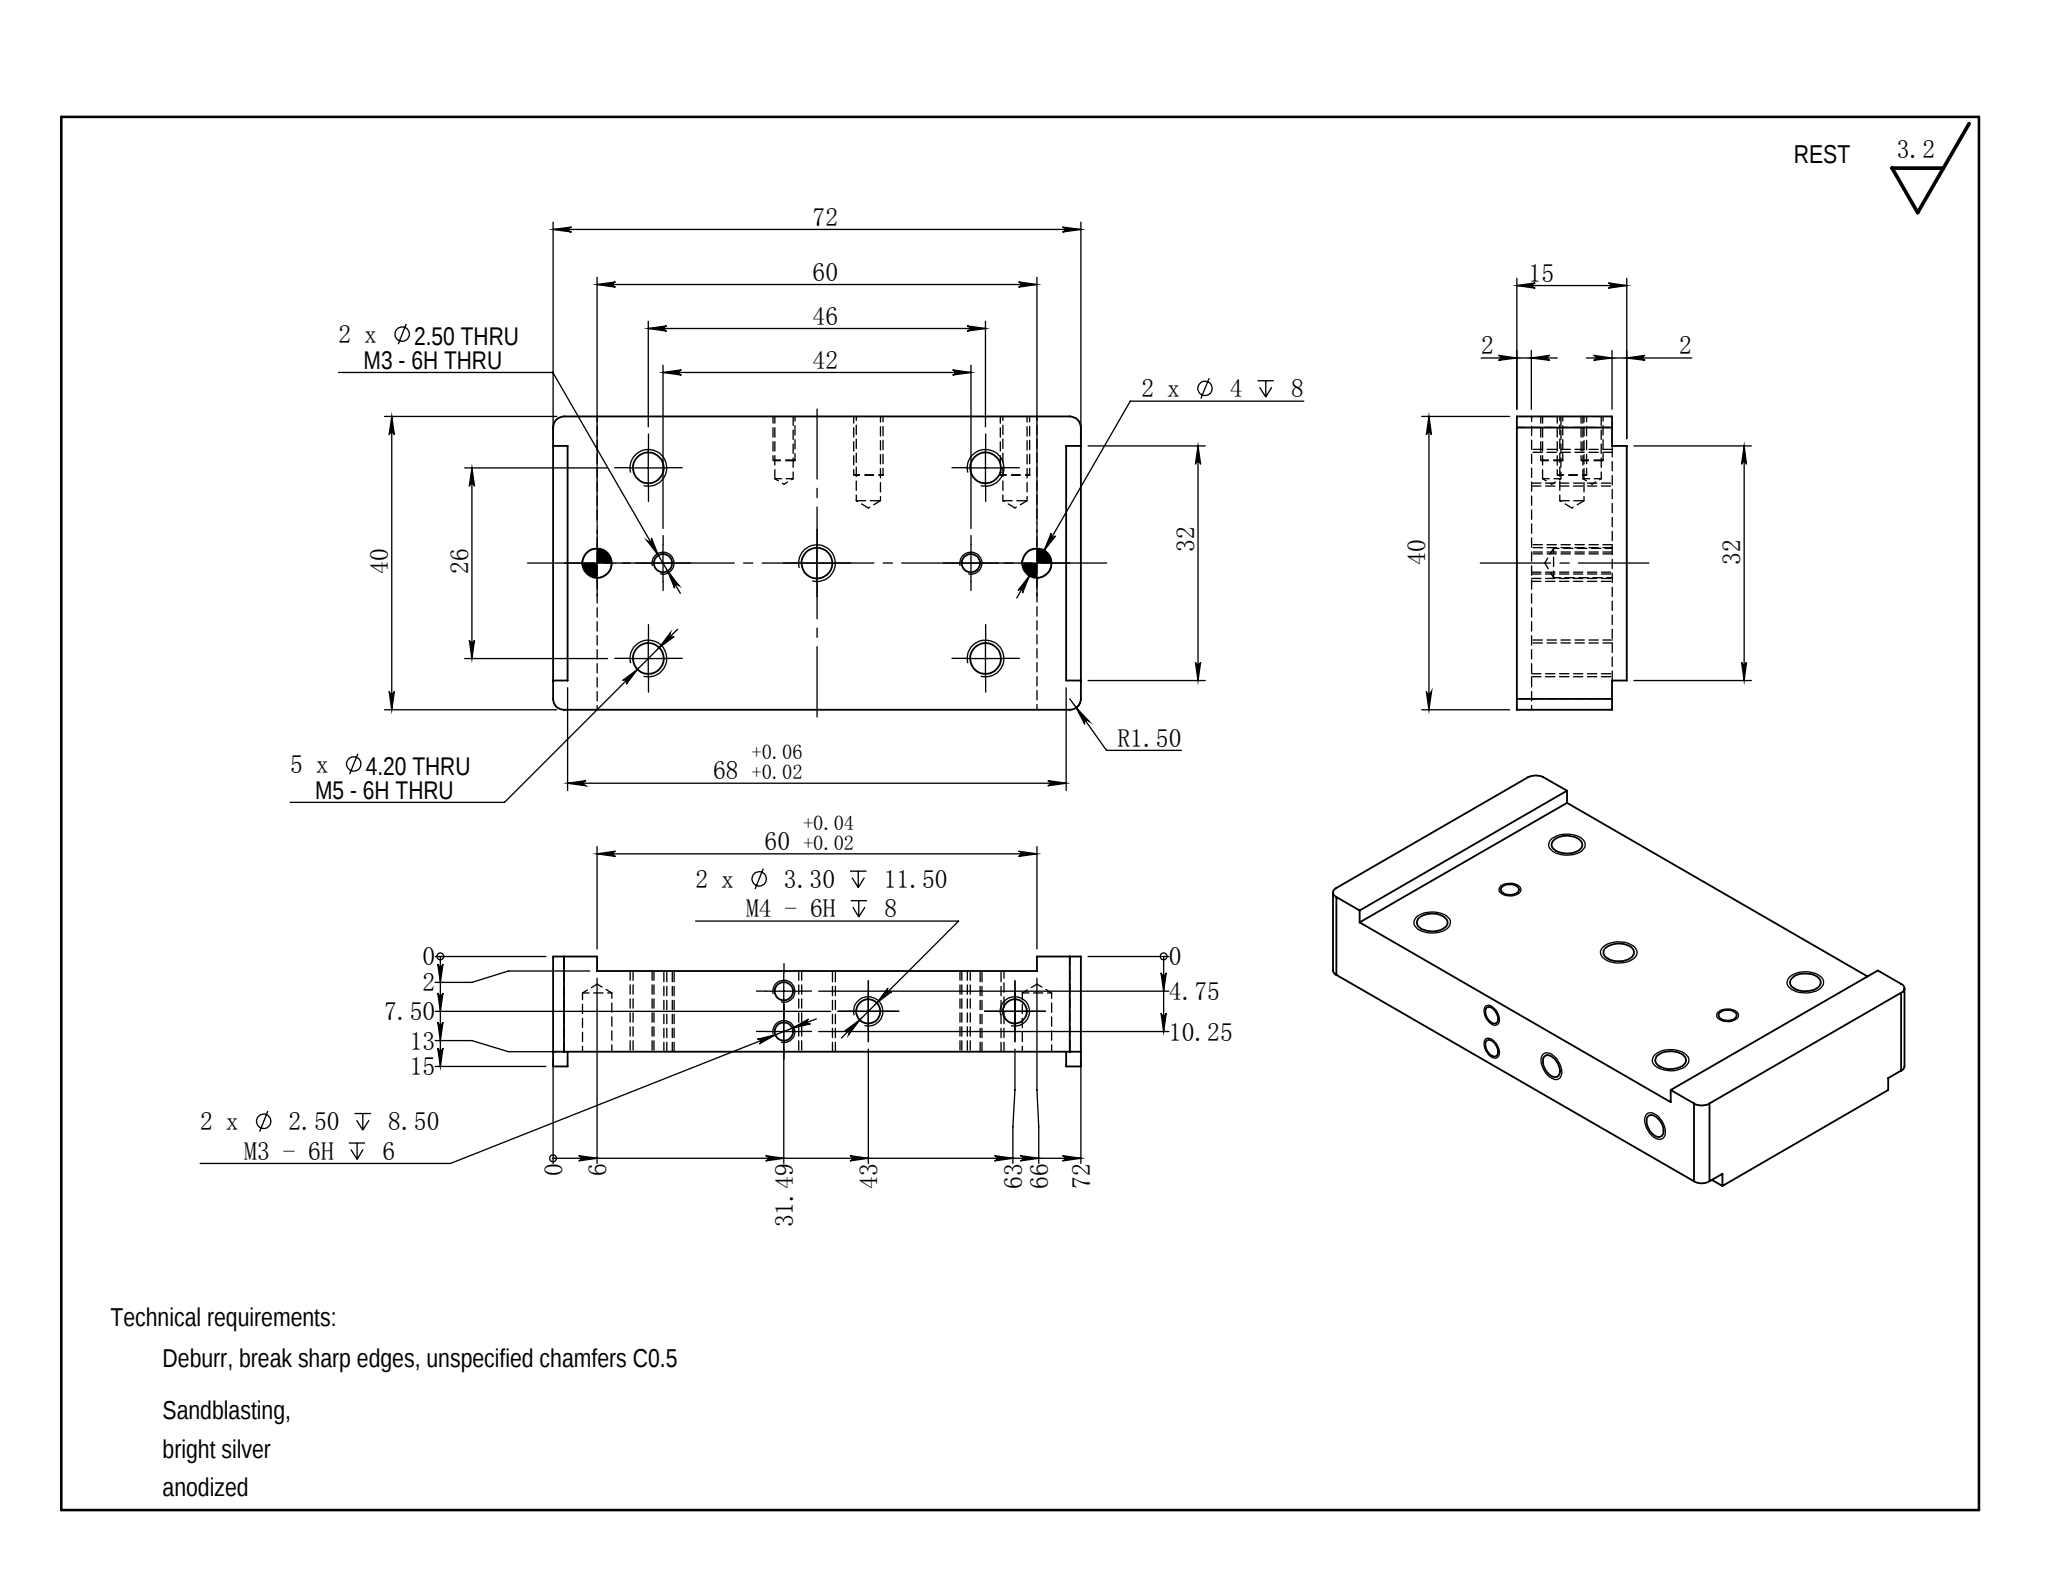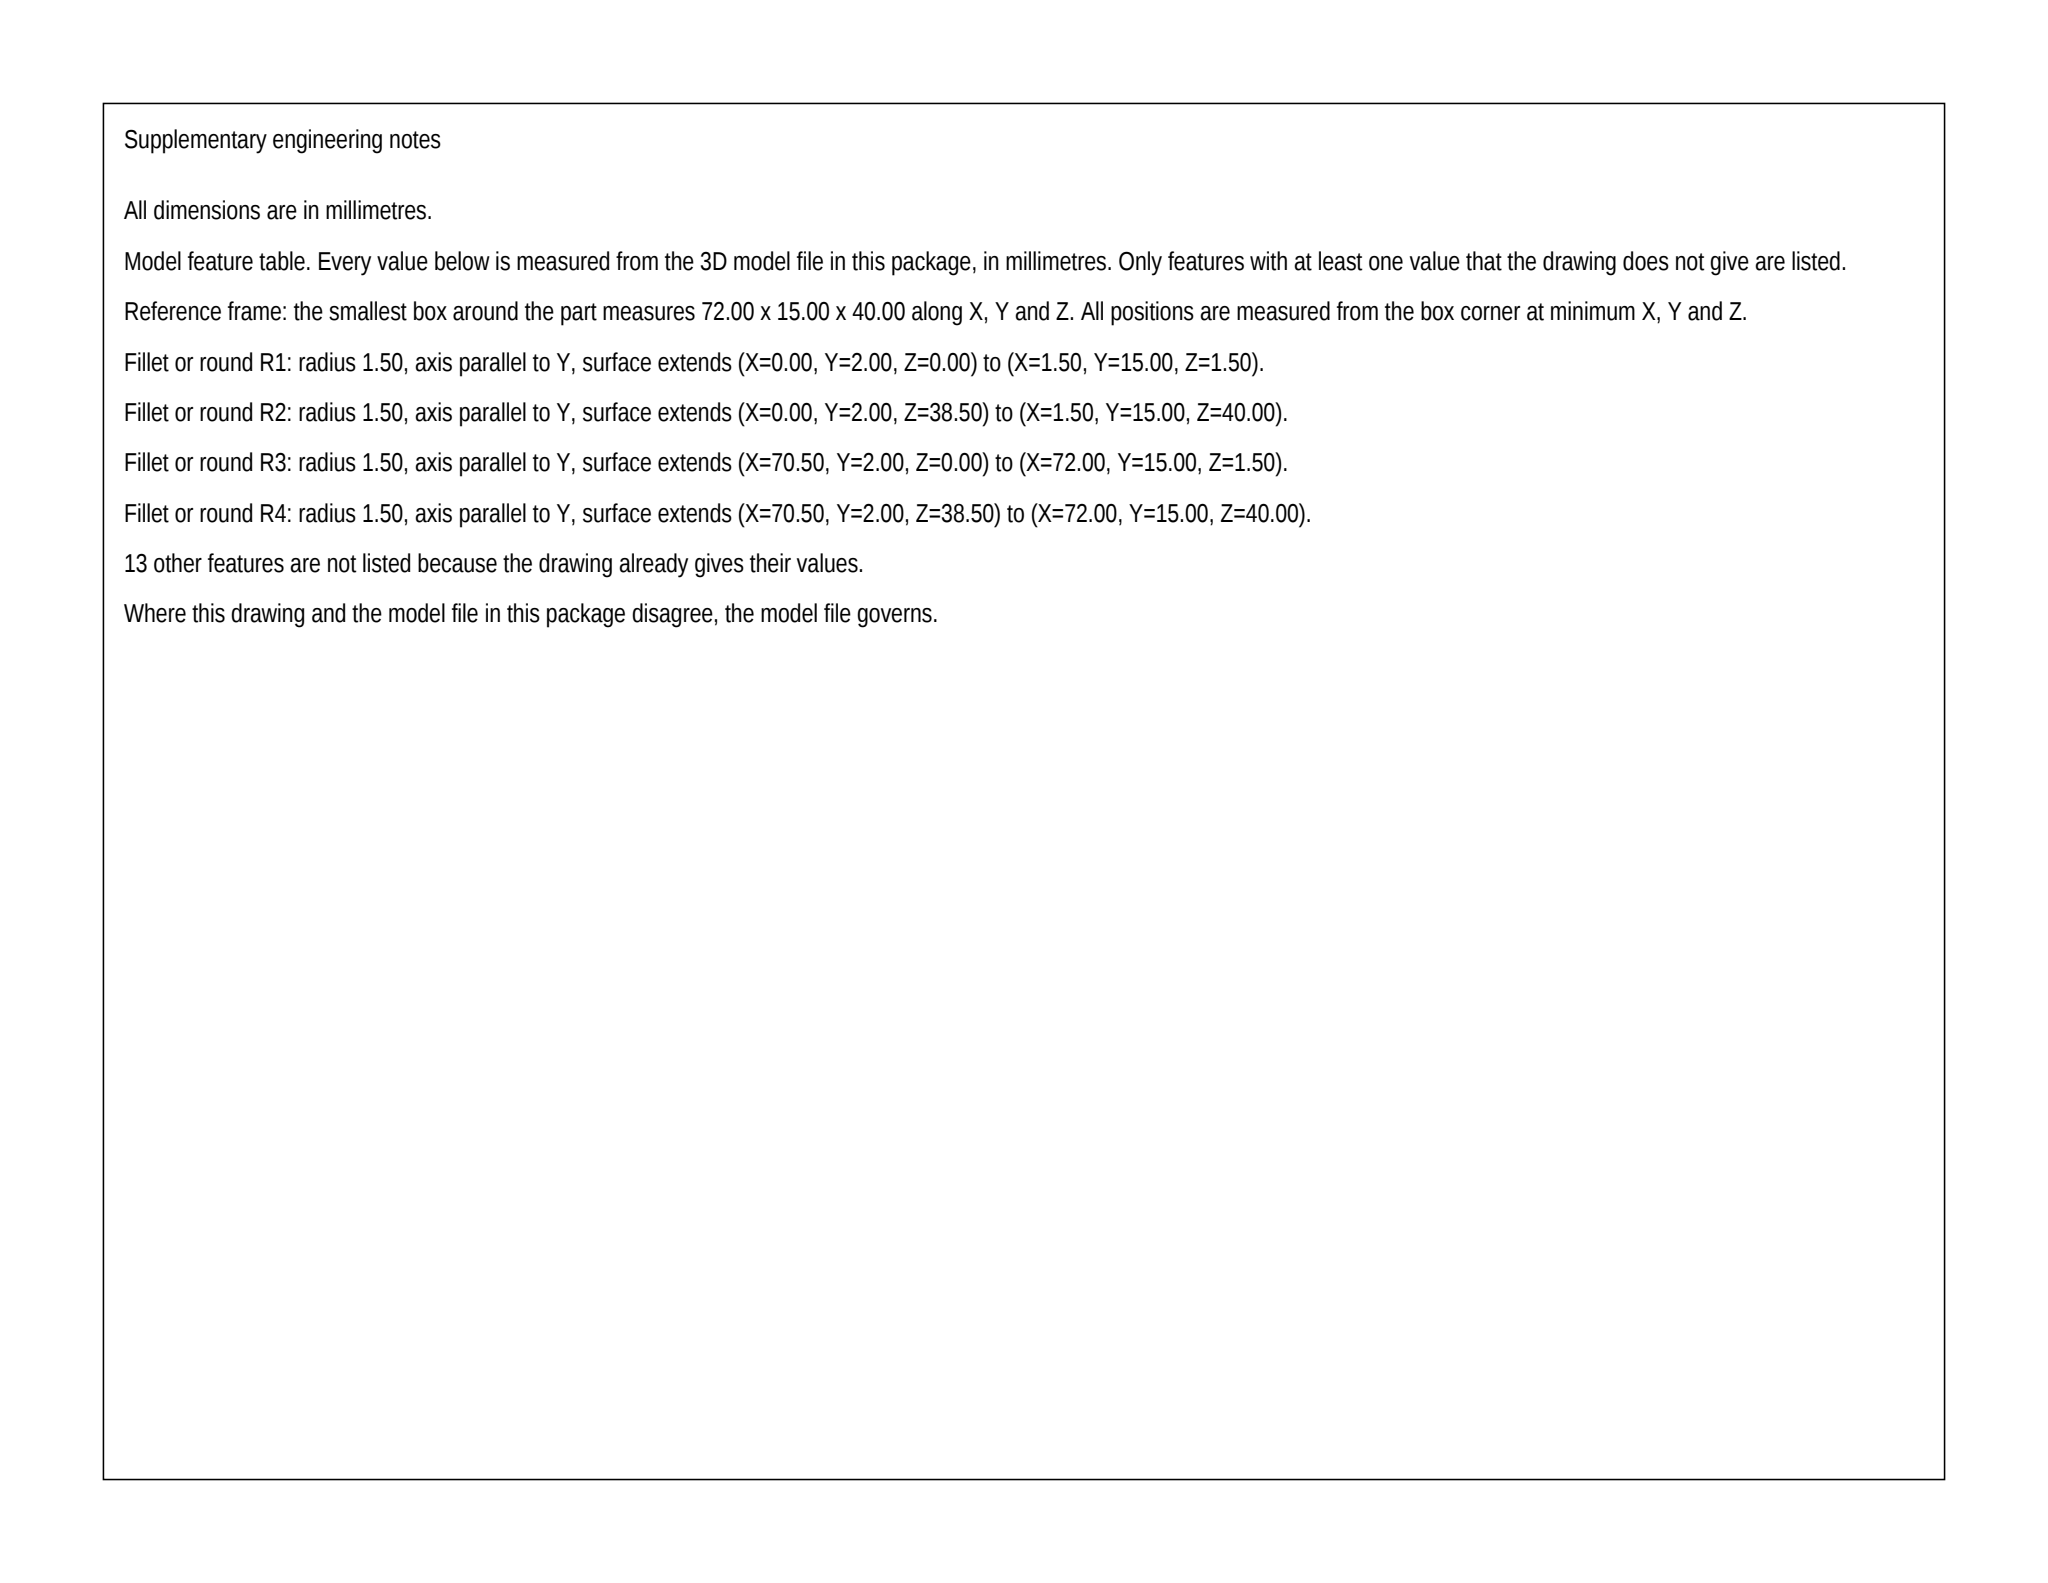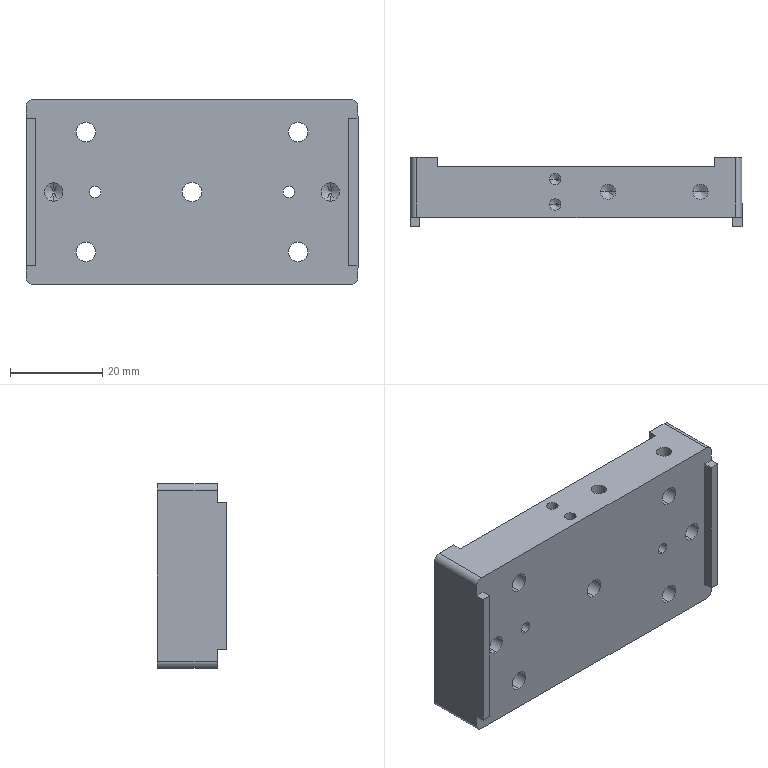Part | SolidWorks | mm | 1 solid | 60 faces | box 72 x 15 x 40 mm | volume 31501 mm3 | cylinder 30 | plane 18 | cone 12 | commonest cylinder face diameters 4.2 x10 2.5 x8 3.3 x4 4 x4 3 x4
Drawing notes:
RECESS 2 DP EA FACE; 32 WIDE BTWN RAILS, RAIL 4 WIDE EA LONG EDGE | from the solid: y planes 0/2 and 13/15 = 2 deep relief both faces; z planes 4 and 36 (2 each) = 32 wide recess, 4 wide rails
TOP RAILS 68 LG (X2-X70); BOT RAILS 60 LG (X6-X66) | from the solid: x planes at 2 and 70 (top rail ends, 68 lg) and at 6 and 66 (bot rail ends, 60 lg); 2 faces each at y=0 and y=15
5 x Ø4.20 THRU M5-6H: 4 ON 46 x 26 PATTERN + 1 AT PLATE CTR | from the solid: Ø4.2 y-axis holes at (x,z)=(13,7),(13,33),(59,7),(59,33) and (36,20); bbox 72x40 so ctr hole = plate center, pattern 46 x 26
2 x Ø4 DP 8 ON HORIZ CL AT X6 & X66 (60 APART) | from the solid: Ø4 y-axis cyl, len 8, at (x,z)=(6,20) and (66,20) from min corner; z=20 = 40/2 centerline
build123d program:
from build123d import *

# Parameters (mm, degrees)
SKETCH1_W                    = 72
SKETCH1_H                    = 40
BOSS_EXTRUDE1_DEPTH          = 15
SKETCH2_W                    = 60
SKETCH2_H                    = 40
CUT_EXTRUDE1_DEPTH           = 2
SKETCH3_W                    = 68
SKETCH3_H                    = 4
CUT_EXTRUDE2_DEPTH           = 56.866
M5_TAPPED_HOLE1_D            = 4.2
M3_TAPPED_HOLE1_D            = 2.5
F_4_0_4_DIAMETER_HOLE1_D     = 4
F_4_0_4_DIAMETER_HOLE1_DEPTH = 8
F_4_0_4_DIAMETER_HOLE1_TIP   = 1.202
FILLET1_R                    = 1.5
M4_TAPPED_HOLE2_D            = 3.3
M4_TAPPED_HOLE2_DEPTH        = 11.5
M4_TAPPED_HOLE2_TIP          = 0.9914
M3_TAPPED_HOLE2_D            = 2.5
M3_TAPPED_HOLE2_DEPTH        = 8.5
M3_TAPPED_HOLE2_TIP          = 0.7511
SKETCH18_OUTSIDE_W           = 90.744
SKETCH18_OUTSIDE_H           = 58.744
SKETCH18_OUTSIDE_W_2         = 72
SKETCH18_OUTSIDE_H_2         = 32
CUT_EXTRUDE3_DEPTH           = 44.186


with BuildPart() as part:
    # Sketch1 → Boss-Extrude1 (new body)
    with BuildSketch(Plane(origin=(0, 0, 0), x_dir=(1, 0, 0), z_dir=(0, 1, 0))):
        Rectangle(SKETCH1_W, SKETCH1_H)
    extrude(amount=BOSS_EXTRUDE1_DEPTH)

    # Sketch2 → Cut-Extrude1 (cut)
    with BuildSketch(Plane(origin=(0, 15, 0), x_dir=(1, 0, 0), z_dir=(0, 1, 0))):
        Rectangle(SKETCH2_W, SKETCH2_H)
    extrude(amount=-CUT_EXTRUDE1_DEPTH, mode=Mode.SUBTRACT)

    # Sketch3 → Cut-Extrude2 (cut, through all)
    with BuildSketch(Plane.XY.offset(20)):
        Rectangle(SKETCH3_W, SKETCH3_H)
    extrude(amount=-CUT_EXTRUDE2_DEPTH, mode=Mode.SUBTRACT)

    # M5 Tapped Hole1 (through all)
    with Locations(Plane(origin=(0, 13, 0), x_dir=(1, 0, 0), z_dir=(0, 1, 0))):
        with Locations((0, 0), (-23, 13), (23, -13), (23, 13), (-23, -13)):
            Hole(M5_TAPPED_HOLE1_D / 2)

    # M3 Tapped Hole1 (through all)
    with Locations(Plane(origin=(0, 13, 0), x_dir=(1, 0, 0), z_dir=(0, 1, 0))):
        with Locations((-21, 0), (21, 0)):
            Hole(M3_TAPPED_HOLE1_D / 2)

    # 4.0 _4_ Diameter Hole1
    with Locations(Plane(origin=(0, 2, 0), x_dir=(-1, 0, 0), z_dir=(0, -1, 0))):
        with Locations((-30, 0), (30, 0)):
            Hole(F_4_0_4_DIAMETER_HOLE1_D / 2, depth=F_4_0_4_DIAMETER_HOLE1_DEPTH)
            with Locations((0, 0, -(F_4_0_4_DIAMETER_HOLE1_DEPTH + F_4_0_4_DIAMETER_HOLE1_TIP / 2))):  # 118° drill point
                Cone(0, F_4_0_4_DIAMETER_HOLE1_D / 2, F_4_0_4_DIAMETER_HOLE1_TIP, mode=Mode.SUBTRACT)

    # Fillet1
    fillet1_edges = [part.edges().sort_by_distance(p)[0] for p in [
        (36, 7.5, 20),
        (-36, 7.5, 20),
        (-36, 7.5, -20),
        (36, 7.5, -20),
    ]]
    fillet(fillet1_edges, radius=FILLET1_R)

    # M4 Tapped Hole2
    with Locations(Plane.XY.offset(20)):
        with Locations((7, 7.5), (27, 7.5)):
            Hole(M4_TAPPED_HOLE2_D / 2, depth=M4_TAPPED_HOLE2_DEPTH)
            with Locations((0, 0, -(M4_TAPPED_HOLE2_DEPTH + M4_TAPPED_HOLE2_TIP / 2))):  # 118° drill point
                Cone(0, M4_TAPPED_HOLE2_D / 2, M4_TAPPED_HOLE2_TIP, mode=Mode.SUBTRACT)

    # M3 Tapped Hole2
    with Locations(Plane.XY.offset(20)):
        with Locations((-4.511, 10.25), (-4.511, 4.75)):
            Hole(M3_TAPPED_HOLE2_D / 2, depth=M3_TAPPED_HOLE2_DEPTH)
            with Locations((0, 0, -(M3_TAPPED_HOLE2_DEPTH + M3_TAPPED_HOLE2_TIP / 2))):  # 118° drill point
                Cone(0, M3_TAPPED_HOLE2_D / 2, M3_TAPPED_HOLE2_TIP, mode=Mode.SUBTRACT)

    # Sketch18 outside → Cut-Extrude3 (cut, through all)
    with BuildSketch(Plane.XZ.offset(-2)):
        Rectangle(SKETCH18_OUTSIDE_W, SKETCH18_OUTSIDE_H)
        Rectangle(SKETCH18_OUTSIDE_W_2, SKETCH18_OUTSIDE_H_2, mode=Mode.SUBTRACT)
    extrude(amount=CUT_EXTRUDE3_DEPTH, mode=Mode.SUBTRACT)


solid = part.part